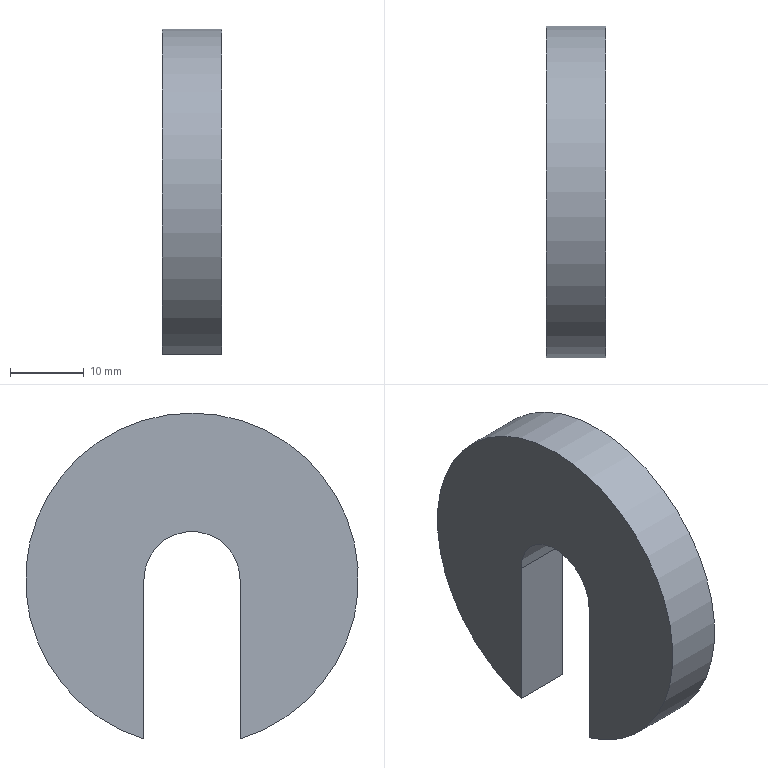Component | NX | SPLIT_WASHER | 1 solid | 6 faces | box 8 x 45 x 44.04 mm | volume 9885 mm3 | plane 4 | cylinder 2 | commonest cylinder face diameters 13 x1 45 x1
STEP:
#1=CARTESIAN_POINT('',(0.,0.,0.));
#2=DIRECTION('',(0.,0.,1.));
#3=DIRECTION('',(1.,0.,0.));
#4=AXIS2_PLACEMENT_3D('',#1,#2,#3);
#5=CARTESIAN_POINT('',(89.,-22.3,112.059));
#6=VERTEX_POINT('',#5);
#7=CARTESIAN_POINT('',(89.,-22.3,133.6));
#8=VERTEX_POINT('',#7);
#9=CARTESIAN_POINT('',(89.,-22.3,112.059));
#10=DIRECTION('',(0.,-0.,1.));
#11=VECTOR('',#10,1.);
#12=LINE('',#9,#11);
#13=CARTESIAN_POINT('',(97.,-22.3,112.059));
#14=DIRECTION('',(0.,-1.,-0.));
#15=DIRECTION('',(0.,0.,-1.));
#16=AXIS2_PLACEMENT_3D('',#13,#14,#15);
#17=PLANE('',#16);
#18=CARTESIAN_POINT('',(0.,-8.));
#19=DIRECTION('',(-1.,0.));
#20=VECTOR('',#19,1.);
#21=LINE('',#18,#20);
#22=(GEOMETRIC_REPRESENTATION_CONTEXT(2)PARAMETRIC_REPRESENTATION_CONTEXT()REPRESENTATION_CONTEXT('',''));
#23=DEFINITIONAL_REPRESENTATION('',(#21),#22);
#24=PCURVE('',#17,#23);
#25=CARTESIAN_POINT('',(89.,-15.8,133.6));
#26=DIRECTION('',(-1.,0.,0.));
#27=DIRECTION('',(0.,-1.,0.));
#28=AXIS2_PLACEMENT_3D('',#25,#26,#27);
#29=PLANE('',#28);
#30=CARTESIAN_POINT('',(6.5,-21.541));
#31=DIRECTION('',(0.,1.));
#32=VECTOR('',#31,1.);
#33=LINE('',#30,#32);
#34=(GEOMETRIC_REPRESENTATION_CONTEXT(2)PARAMETRIC_REPRESENTATION_CONTEXT()REPRESENTATION_CONTEXT('',''));
#35=DEFINITIONAL_REPRESENTATION('',(#33),#34);
#36=PCURVE('',#29,#35);
#37=SURFACE_CURVE('',#12,(#24,#36),.PCURVE_S1.);
#38=EDGE_CURVE('',#6,#8,#37,.T.);
#39=ORIENTED_EDGE('',*,*,#38,.T.);
#40=CARTESIAN_POINT('',(97.,-22.3,133.6));
#41=VERTEX_POINT('',#40);
#42=CARTESIAN_POINT('',(97.,-22.3,133.6));
#43=DIRECTION('',(-1.,0.,0.));
#44=VECTOR('',#43,1.);
#45=LINE('',#42,#44);
#46=CARTESIAN_POINT('',(-21.541,0.));
#47=DIRECTION('',(0.,-1.));
#48=VECTOR('',#47,1.);
#49=LINE('',#46,#48);
#50=(GEOMETRIC_REPRESENTATION_CONTEXT(2)PARAMETRIC_REPRESENTATION_CONTEXT()REPRESENTATION_CONTEXT('',''));
#51=DEFINITIONAL_REPRESENTATION('',(#49),#50);
#52=PCURVE('',#17,#51);
#53=CARTESIAN_POINT('',(97.,-15.8,133.6));
#54=DIRECTION('',(-1.,0.,0.));
#55=DIRECTION('',(0.,-1.,0.));
#56=AXIS2_PLACEMENT_3D('',#53,#54,#55);
#57=CYLINDRICAL_SURFACE('',#56,6.5);
#58=CARTESIAN_POINT('',(0.,0.));
#59=DIRECTION('',(0.,1.));
#60=VECTOR('',#59,1.);
#61=LINE('',#58,#60);
#62=(GEOMETRIC_REPRESENTATION_CONTEXT(2)PARAMETRIC_REPRESENTATION_CONTEXT()REPRESENTATION_CONTEXT('',''));
#63=DEFINITIONAL_REPRESENTATION('',(#61),#62);
#64=PCURVE('',#57,#63);
#65=SURFACE_CURVE('',#45,(#52,#64),.PCURVE_S1.);
#66=EDGE_CURVE('',#41,#8,#65,.T.);
#67=ORIENTED_EDGE('',*,*,#66,.F.);
#68=CARTESIAN_POINT('',(97.,-22.3,112.059));
#69=VERTEX_POINT('',#68);
#70=CARTESIAN_POINT('',(97.,-22.3,112.059));
#71=DIRECTION('',(0.,-0.,1.));
#72=VECTOR('',#71,1.);
#73=LINE('',#70,#72);
#74=CARTESIAN_POINT('',(0.,0.));
#75=DIRECTION('',(-1.,0.));
#76=VECTOR('',#75,1.);
#77=LINE('',#74,#76);
#78=(GEOMETRIC_REPRESENTATION_CONTEXT(2)PARAMETRIC_REPRESENTATION_CONTEXT()REPRESENTATION_CONTEXT('',''));
#79=DEFINITIONAL_REPRESENTATION('',(#77),#78);
#80=PCURVE('',#17,#79);
#81=CARTESIAN_POINT('',(97.,-15.8,133.6));
#82=DIRECTION('',(-1.,0.,0.));
#83=DIRECTION('',(0.,-1.,0.));
#84=AXIS2_PLACEMENT_3D('',#81,#82,#83);
#85=PLANE('',#84);
#86=CARTESIAN_POINT('',(6.5,-21.541));
#87=DIRECTION('',(0.,1.));
#88=VECTOR('',#87,1.);
#89=LINE('',#86,#88);
#90=(GEOMETRIC_REPRESENTATION_CONTEXT(2)PARAMETRIC_REPRESENTATION_CONTEXT()REPRESENTATION_CONTEXT('',''));
#91=DEFINITIONAL_REPRESENTATION('',(#89),#90);
#92=PCURVE('',#85,#91);
#93=SURFACE_CURVE('',#73,(#80,#92),.PCURVE_S1.);
#94=EDGE_CURVE('',#69,#41,#93,.T.);
#95=ORIENTED_EDGE('',*,*,#94,.F.);
#96=CARTESIAN_POINT('',(97.,-22.3,112.059));
#97=DIRECTION('',(-1.,0.,0.));
#98=VECTOR('',#97,1.);
#99=LINE('',#96,#98);
#100=CARTESIAN_POINT('',(0.,0.));
#101=DIRECTION('',(0.,-1.));
#102=VECTOR('',#101,1.);
#103=LINE('',#100,#102);
#104=(GEOMETRIC_REPRESENTATION_CONTEXT(2)PARAMETRIC_REPRESENTATION_CONTEXT()REPRESENTATION_CONTEXT('',''));
#105=DEFINITIONAL_REPRESENTATION('',(#103),#104);
#106=PCURVE('',#17,#105);
#107=CARTESIAN_POINT('',(97.,-15.8,133.6));
#108=DIRECTION('',(-1.,0.,0.));
#109=DIRECTION('',(0.,-1.,0.));
#110=AXIS2_PLACEMENT_3D('',#107,#108,#109);
#111=CYLINDRICAL_SURFACE('',#110,22.5);
#112=CARTESIAN_POINT('',(-1.278,0.));
#113=DIRECTION('',(0.,1.));
#114=VECTOR('',#113,1.);
#115=LINE('',#112,#114);
#116=(GEOMETRIC_REPRESENTATION_CONTEXT(2)PARAMETRIC_REPRESENTATION_CONTEXT()REPRESENTATION_CONTEXT('',''));
#117=DEFINITIONAL_REPRESENTATION('',(#115),#116);
#118=PCURVE('',#111,#117);
#119=SURFACE_CURVE('',#99,(#106,#118),.PCURVE_S1.);
#120=EDGE_CURVE('',#69,#6,#119,.T.);
#121=ORIENTED_EDGE('',*,*,#120,.T.);
#122=EDGE_LOOP('',(#39,#67,#95,#121));
#123=FACE_BOUND('',#122,.T.);
#124=ADVANCED_FACE('',(#123),#17,.F.);
#125=ORIENTED_EDGE('',*,*,#66,.F.);
#126=CARTESIAN_POINT('',(97.,-9.3,133.6));
#127=VERTEX_POINT('',#126);
#128=CARTESIAN_POINT('',(97.,-15.8,133.6));
#129=DIRECTION('',(-1.,0.,0.));
#130=DIRECTION('',(0.,1.,0.));
#131=AXIS2_PLACEMENT_3D('',#128,#129,#130);
#132=CIRCLE('',#131,6.5);
#133=CARTESIAN_POINT('',(-3.142,0.));
#134=DIRECTION('',(1.,0.));
#135=VECTOR('',#134,1.);
#136=LINE('',#133,#135);
#137=(GEOMETRIC_REPRESENTATION_CONTEXT(2)PARAMETRIC_REPRESENTATION_CONTEXT()REPRESENTATION_CONTEXT('',''));
#138=DEFINITIONAL_REPRESENTATION('',(#136),#137);
#139=PCURVE('',#57,#138);
#140=CARTESIAN_POINT('',(0.,0.));
#141=DIRECTION('',(-1.,0.));
#142=AXIS2_PLACEMENT_2D('',#140,#141);
#143=CIRCLE('',#142,6.5);
#144=(GEOMETRIC_REPRESENTATION_CONTEXT(2)PARAMETRIC_REPRESENTATION_CONTEXT()REPRESENTATION_CONTEXT('',''));
#145=DEFINITIONAL_REPRESENTATION('',(#143),#144);
#146=PCURVE('',#85,#145);
#147=SURFACE_CURVE('',#132,(#139,#146),.PCURVE_S1.);
#148=EDGE_CURVE('',#41,#127,#147,.T.);
#149=ORIENTED_EDGE('',*,*,#148,.T.);
#150=CARTESIAN_POINT('',(89.,-9.3,133.6));
#151=VERTEX_POINT('',#150);
#152=CARTESIAN_POINT('',(97.,-9.3,133.6));
#153=DIRECTION('',(-1.,0.,0.));
#154=VECTOR('',#153,1.);
#155=LINE('',#152,#154);
#156=CARTESIAN_POINT('',(3.142,0.));
#157=DIRECTION('',(0.,1.));
#158=VECTOR('',#157,1.);
#159=LINE('',#156,#158);
#160=(GEOMETRIC_REPRESENTATION_CONTEXT(2)PARAMETRIC_REPRESENTATION_CONTEXT()REPRESENTATION_CONTEXT('',''));
#161=DEFINITIONAL_REPRESENTATION('',(#159),#160);
#162=PCURVE('',#57,#161);
#163=CARTESIAN_POINT('',(97.,-9.3,133.6));
#164=DIRECTION('',(0.,1.,0.));
#165=DIRECTION('',(0.,-0.,1.));
#166=AXIS2_PLACEMENT_3D('',#163,#164,#165);
#167=PLANE('',#166);
#168=CARTESIAN_POINT('',(0.,0.));
#169=DIRECTION('',(0.,-1.));
#170=VECTOR('',#169,1.);
#171=LINE('',#168,#170);
#172=(GEOMETRIC_REPRESENTATION_CONTEXT(2)PARAMETRIC_REPRESENTATION_CONTEXT()REPRESENTATION_CONTEXT('',''));
#173=DEFINITIONAL_REPRESENTATION('',(#171),#172);
#174=PCURVE('',#167,#173);
#175=SURFACE_CURVE('',#155,(#162,#174),.PCURVE_S1.);
#176=EDGE_CURVE('',#127,#151,#175,.T.);
#177=ORIENTED_EDGE('',*,*,#176,.T.);
#178=CARTESIAN_POINT('',(89.,-15.8,133.6));
#179=DIRECTION('',(-1.,0.,0.));
#180=DIRECTION('',(0.,1.,0.));
#181=AXIS2_PLACEMENT_3D('',#178,#179,#180);
#182=CIRCLE('',#181,6.5);
#183=CARTESIAN_POINT('',(-3.142,8.));
#184=DIRECTION('',(1.,0.));
#185=VECTOR('',#184,1.);
#186=LINE('',#183,#185);
#187=(GEOMETRIC_REPRESENTATION_CONTEXT(2)PARAMETRIC_REPRESENTATION_CONTEXT()REPRESENTATION_CONTEXT('',''));
#188=DEFINITIONAL_REPRESENTATION('',(#186),#187);
#189=PCURVE('',#57,#188);
#190=CARTESIAN_POINT('',(0.,0.));
#191=DIRECTION('',(-1.,0.));
#192=AXIS2_PLACEMENT_2D('',#190,#191);
#193=CIRCLE('',#192,6.5);
#194=(GEOMETRIC_REPRESENTATION_CONTEXT(2)PARAMETRIC_REPRESENTATION_CONTEXT()REPRESENTATION_CONTEXT('',''));
#195=DEFINITIONAL_REPRESENTATION('',(#193),#194);
#196=PCURVE('',#29,#195);
#197=SURFACE_CURVE('',#182,(#189,#196),.PCURVE_S1.);
#198=EDGE_CURVE('',#8,#151,#197,.T.);
#199=ORIENTED_EDGE('',*,*,#198,.F.);
#200=EDGE_LOOP('',(#125,#149,#177,#199));
#201=FACE_BOUND('',#200,.F.);
#202=ADVANCED_FACE('',(#201),#57,.F.);
#203=CARTESIAN_POINT('',(89.,-9.3,112.059));
#204=VERTEX_POINT('',#203);
#205=CARTESIAN_POINT('',(89.,-9.3,133.6));
#206=DIRECTION('',(0.,0.,-1.));
#207=VECTOR('',#206,1.);
#208=LINE('',#205,#207);
#209=CARTESIAN_POINT('',(0.,-8.));
#210=DIRECTION('',(-1.,0.));
#211=VECTOR('',#210,1.);
#212=LINE('',#209,#211);
#213=(GEOMETRIC_REPRESENTATION_CONTEXT(2)PARAMETRIC_REPRESENTATION_CONTEXT()REPRESENTATION_CONTEXT('',''));
#214=DEFINITIONAL_REPRESENTATION('',(#212),#213);
#215=PCURVE('',#167,#214);
#216=CARTESIAN_POINT('',(-6.5,0.));
#217=DIRECTION('',(-0.,-1.));
#218=VECTOR('',#217,1.);
#219=LINE('',#216,#218);
#220=(GEOMETRIC_REPRESENTATION_CONTEXT(2)PARAMETRIC_REPRESENTATION_CONTEXT()REPRESENTATION_CONTEXT('',''));
#221=DEFINITIONAL_REPRESENTATION('',(#219),#220);
#222=PCURVE('',#29,#221);
#223=SURFACE_CURVE('',#208,(#215,#222),.PCURVE_S1.);
#224=EDGE_CURVE('',#151,#204,#223,.T.);
#225=ORIENTED_EDGE('',*,*,#224,.T.);
#226=CARTESIAN_POINT('',(97.,-9.3,112.059));
#227=VERTEX_POINT('',#226);
#228=CARTESIAN_POINT('',(97.,-9.3,112.059));
#229=DIRECTION('',(-1.,0.,0.));
#230=VECTOR('',#229,1.);
#231=LINE('',#228,#230);
#232=CARTESIAN_POINT('',(-21.541,0.));
#233=DIRECTION('',(0.,-1.));
#234=VECTOR('',#233,1.);
#235=LINE('',#232,#234);
#236=(GEOMETRIC_REPRESENTATION_CONTEXT(2)PARAMETRIC_REPRESENTATION_CONTEXT()REPRESENTATION_CONTEXT('',''));
#237=DEFINITIONAL_REPRESENTATION('',(#235),#236);
#238=PCURVE('',#167,#237);
#239=CARTESIAN_POINT('',(4.419,0.));
#240=DIRECTION('',(0.,1.));
#241=VECTOR('',#240,1.);
#242=LINE('',#239,#241);
#243=(GEOMETRIC_REPRESENTATION_CONTEXT(2)PARAMETRIC_REPRESENTATION_CONTEXT()REPRESENTATION_CONTEXT('',''));
#244=DEFINITIONAL_REPRESENTATION('',(#242),#243);
#245=PCURVE('',#111,#244);
#246=SURFACE_CURVE('',#231,(#238,#245),.PCURVE_S1.);
#247=EDGE_CURVE('',#227,#204,#246,.T.);
#248=ORIENTED_EDGE('',*,*,#247,.F.);
#249=CARTESIAN_POINT('',(97.,-9.3,133.6));
#250=DIRECTION('',(0.,0.,-1.));
#251=VECTOR('',#250,1.);
#252=LINE('',#249,#251);
#253=CARTESIAN_POINT('',(0.,0.));
#254=DIRECTION('',(-1.,0.));
#255=VECTOR('',#254,1.);
#256=LINE('',#253,#255);
#257=(GEOMETRIC_REPRESENTATION_CONTEXT(2)PARAMETRIC_REPRESENTATION_CONTEXT()REPRESENTATION_CONTEXT('',''));
#258=DEFINITIONAL_REPRESENTATION('',(#256),#257);
#259=PCURVE('',#167,#258);
#260=CARTESIAN_POINT('',(-6.5,0.));
#261=DIRECTION('',(-0.,-1.));
#262=VECTOR('',#261,1.);
#263=LINE('',#260,#262);
#264=(GEOMETRIC_REPRESENTATION_CONTEXT(2)PARAMETRIC_REPRESENTATION_CONTEXT()REPRESENTATION_CONTEXT('',''));
#265=DEFINITIONAL_REPRESENTATION('',(#263),#264);
#266=PCURVE('',#85,#265);
#267=SURFACE_CURVE('',#252,(#259,#266),.PCURVE_S1.);
#268=EDGE_CURVE('',#127,#227,#267,.T.);
#269=ORIENTED_EDGE('',*,*,#268,.F.);
#270=ORIENTED_EDGE('',*,*,#176,.T.);
#271=EDGE_LOOP('',(#225,#248,#269,#270));
#272=FACE_BOUND('',#271,.T.);
#273=ADVANCED_FACE('',(#272),#167,.F.);
#274=CARTESIAN_POINT('',(89.,-15.8,133.6));
#275=DIRECTION('',(1.,0.,0.));
#276=DIRECTION('',(0.,1.,0.));
#277=AXIS2_PLACEMENT_3D('',#274,#275,#276);
#278=CIRCLE('',#277,22.5);
#279=CARTESIAN_POINT('',(9.425,8.));
#280=DIRECTION('',(-1.,0.));
#281=VECTOR('',#280,1.);
#282=LINE('',#279,#281);
#283=(GEOMETRIC_REPRESENTATION_CONTEXT(2)PARAMETRIC_REPRESENTATION_CONTEXT()REPRESENTATION_CONTEXT('',''));
#284=DEFINITIONAL_REPRESENTATION('',(#282),#283);
#285=PCURVE('',#111,#284);
#286=CARTESIAN_POINT('',(-22.5,0.));
#287=CARTESIAN_POINT('',(-22.5,38.971));
#288=CARTESIAN_POINT('',(11.25,19.486));
#289=CARTESIAN_POINT('',(45.,0.));
#290=CARTESIAN_POINT('',(11.25,-19.486));
#291=CARTESIAN_POINT('',(-22.5,-38.971));
#292=CARTESIAN_POINT('',(-22.5,0.));
#293=(BOUNDED_CURVE()B_SPLINE_CURVE(2,(#286,#287,#288,#289,#290,#291,#292),.UNSPECIFIED.,.T.,.F.)B_SPLINE_CURVE_WITH_KNOTS((1,2,2,2,2,1),(-2.094,0.,2.094,4.189,6.283,8.378),.UNSPECIFIED.)CURVE()GEOMETRIC_REPRESENTATION_ITEM()RATIONAL_B_SPLINE_CURVE((1.,0.5,1.,0.5,1.,0.5,1.))REPRESENTATION_ITEM(''));
#294=(GEOMETRIC_REPRESENTATION_CONTEXT(2)PARAMETRIC_REPRESENTATION_CONTEXT()REPRESENTATION_CONTEXT('',''));
#295=DEFINITIONAL_REPRESENTATION('',(#293),#294);
#296=PCURVE('',#29,#295);
#297=SURFACE_CURVE('',#278,(#285,#296),.PCURVE_S1.);
#298=EDGE_CURVE('',#204,#6,#297,.T.);
#299=ORIENTED_EDGE('',*,*,#298,.T.);
#300=ORIENTED_EDGE('',*,*,#120,.F.);
#301=CARTESIAN_POINT('',(97.,-15.8,133.6));
#302=DIRECTION('',(1.,0.,0.));
#303=DIRECTION('',(0.,1.,0.));
#304=AXIS2_PLACEMENT_3D('',#301,#302,#303);
#305=CIRCLE('',#304,22.5);
#306=CARTESIAN_POINT('',(9.425,0.));
#307=DIRECTION('',(-1.,0.));
#308=VECTOR('',#307,1.);
#309=LINE('',#306,#308);
#310=(GEOMETRIC_REPRESENTATION_CONTEXT(2)PARAMETRIC_REPRESENTATION_CONTEXT()REPRESENTATION_CONTEXT('',''));
#311=DEFINITIONAL_REPRESENTATION('',(#309),#310);
#312=PCURVE('',#111,#311);
#313=CARTESIAN_POINT('',(-22.5,0.));
#314=CARTESIAN_POINT('',(-22.5,38.971));
#315=CARTESIAN_POINT('',(11.25,19.486));
#316=CARTESIAN_POINT('',(45.,0.));
#317=CARTESIAN_POINT('',(11.25,-19.486));
#318=CARTESIAN_POINT('',(-22.5,-38.971));
#319=CARTESIAN_POINT('',(-22.5,0.));
#320=(BOUNDED_CURVE()B_SPLINE_CURVE(2,(#313,#314,#315,#316,#317,#318,#319),.UNSPECIFIED.,.T.,.F.)B_SPLINE_CURVE_WITH_KNOTS((1,2,2,2,2,1),(-2.094,0.,2.094,4.189,6.283,8.378),.UNSPECIFIED.)CURVE()GEOMETRIC_REPRESENTATION_ITEM()RATIONAL_B_SPLINE_CURVE((1.,0.5,1.,0.5,1.,0.5,1.))REPRESENTATION_ITEM(''));
#321=(GEOMETRIC_REPRESENTATION_CONTEXT(2)PARAMETRIC_REPRESENTATION_CONTEXT()REPRESENTATION_CONTEXT('',''));
#322=DEFINITIONAL_REPRESENTATION('',(#320),#321);
#323=PCURVE('',#85,#322);
#324=SURFACE_CURVE('',#305,(#312,#323),.PCURVE_S1.);
#325=EDGE_CURVE('',#227,#69,#324,.T.);
#326=ORIENTED_EDGE('',*,*,#325,.F.);
#327=ORIENTED_EDGE('',*,*,#247,.T.);
#328=EDGE_LOOP('',(#299,#300,#326,#327));
#329=FACE_BOUND('',#328,.T.);
#330=ADVANCED_FACE('',(#329),#111,.T.);
#331=ORIENTED_EDGE('',*,*,#94,.T.);
#332=ORIENTED_EDGE('',*,*,#148,.T.);
#333=ORIENTED_EDGE('',*,*,#268,.T.);
#334=ORIENTED_EDGE('',*,*,#325,.T.);
#335=EDGE_LOOP('',(#331,#332,#333,#334));
#336=FACE_BOUND('',#335,.T.);
#337=ADVANCED_FACE('',(#336),#85,.F.);
#338=ORIENTED_EDGE('',*,*,#38,.F.);
#339=ORIENTED_EDGE('',*,*,#298,.F.);
#340=ORIENTED_EDGE('',*,*,#224,.F.);
#341=ORIENTED_EDGE('',*,*,#198,.F.);
#342=EDGE_LOOP('',(#338,#339,#340,#341));
#343=FACE_BOUND('',#342,.T.);
#344=ADVANCED_FACE('',(#343),#29,.T.);
#345=CLOSED_SHELL('',(#124,#202,#273,#330,#337,#344));
#346=MANIFOLD_SOLID_BREP('',#345);
#347=(LENGTH_UNIT()NAMED_UNIT(*)SI_UNIT(.MILLI.,.METRE.));
#348=UNCERTAINTY_MEASURE_WITH_UNIT(LENGTH_MEASURE(0.0000001),#347,'','');
#349=(NAMED_UNIT(*)PLANE_ANGLE_UNIT()SI_UNIT($,.RADIAN.));
#350=(NAMED_UNIT(*)SI_UNIT($,.STERADIAN.)SOLID_ANGLE_UNIT());
#351=(GEOMETRIC_REPRESENTATION_CONTEXT(3)GLOBAL_UNCERTAINTY_ASSIGNED_CONTEXT((#348))GLOBAL_UNIT_ASSIGNED_CONTEXT((#347,#349,#350))REPRESENTATION_CONTEXT('',''));
#352=ADVANCED_BREP_SHAPE_REPRESENTATION('',(#4,#346),#351);